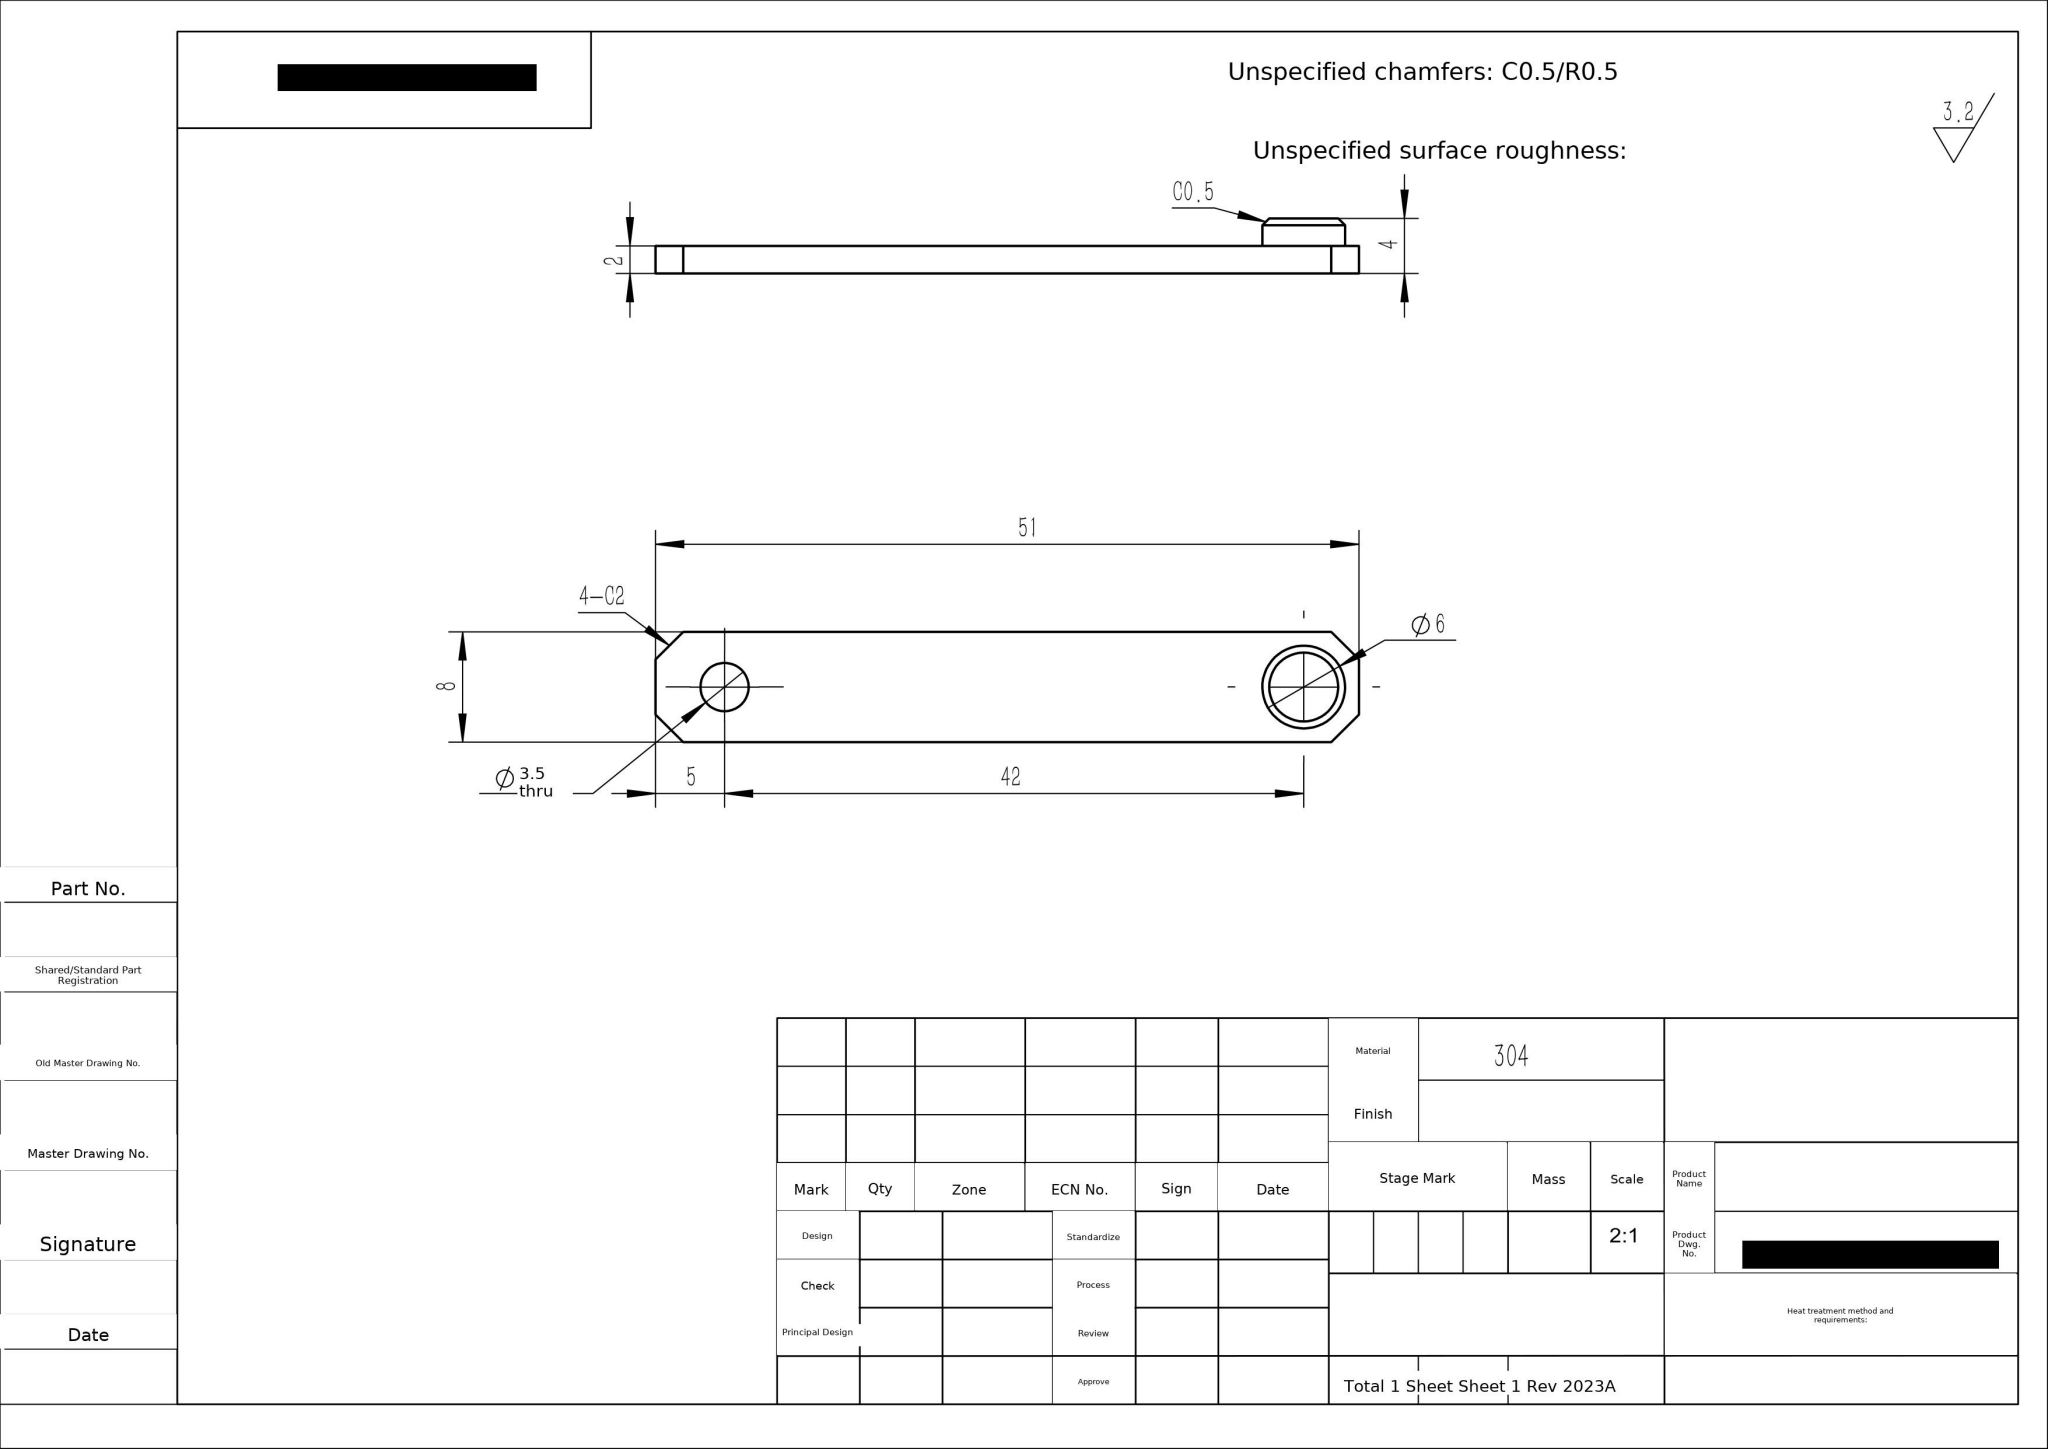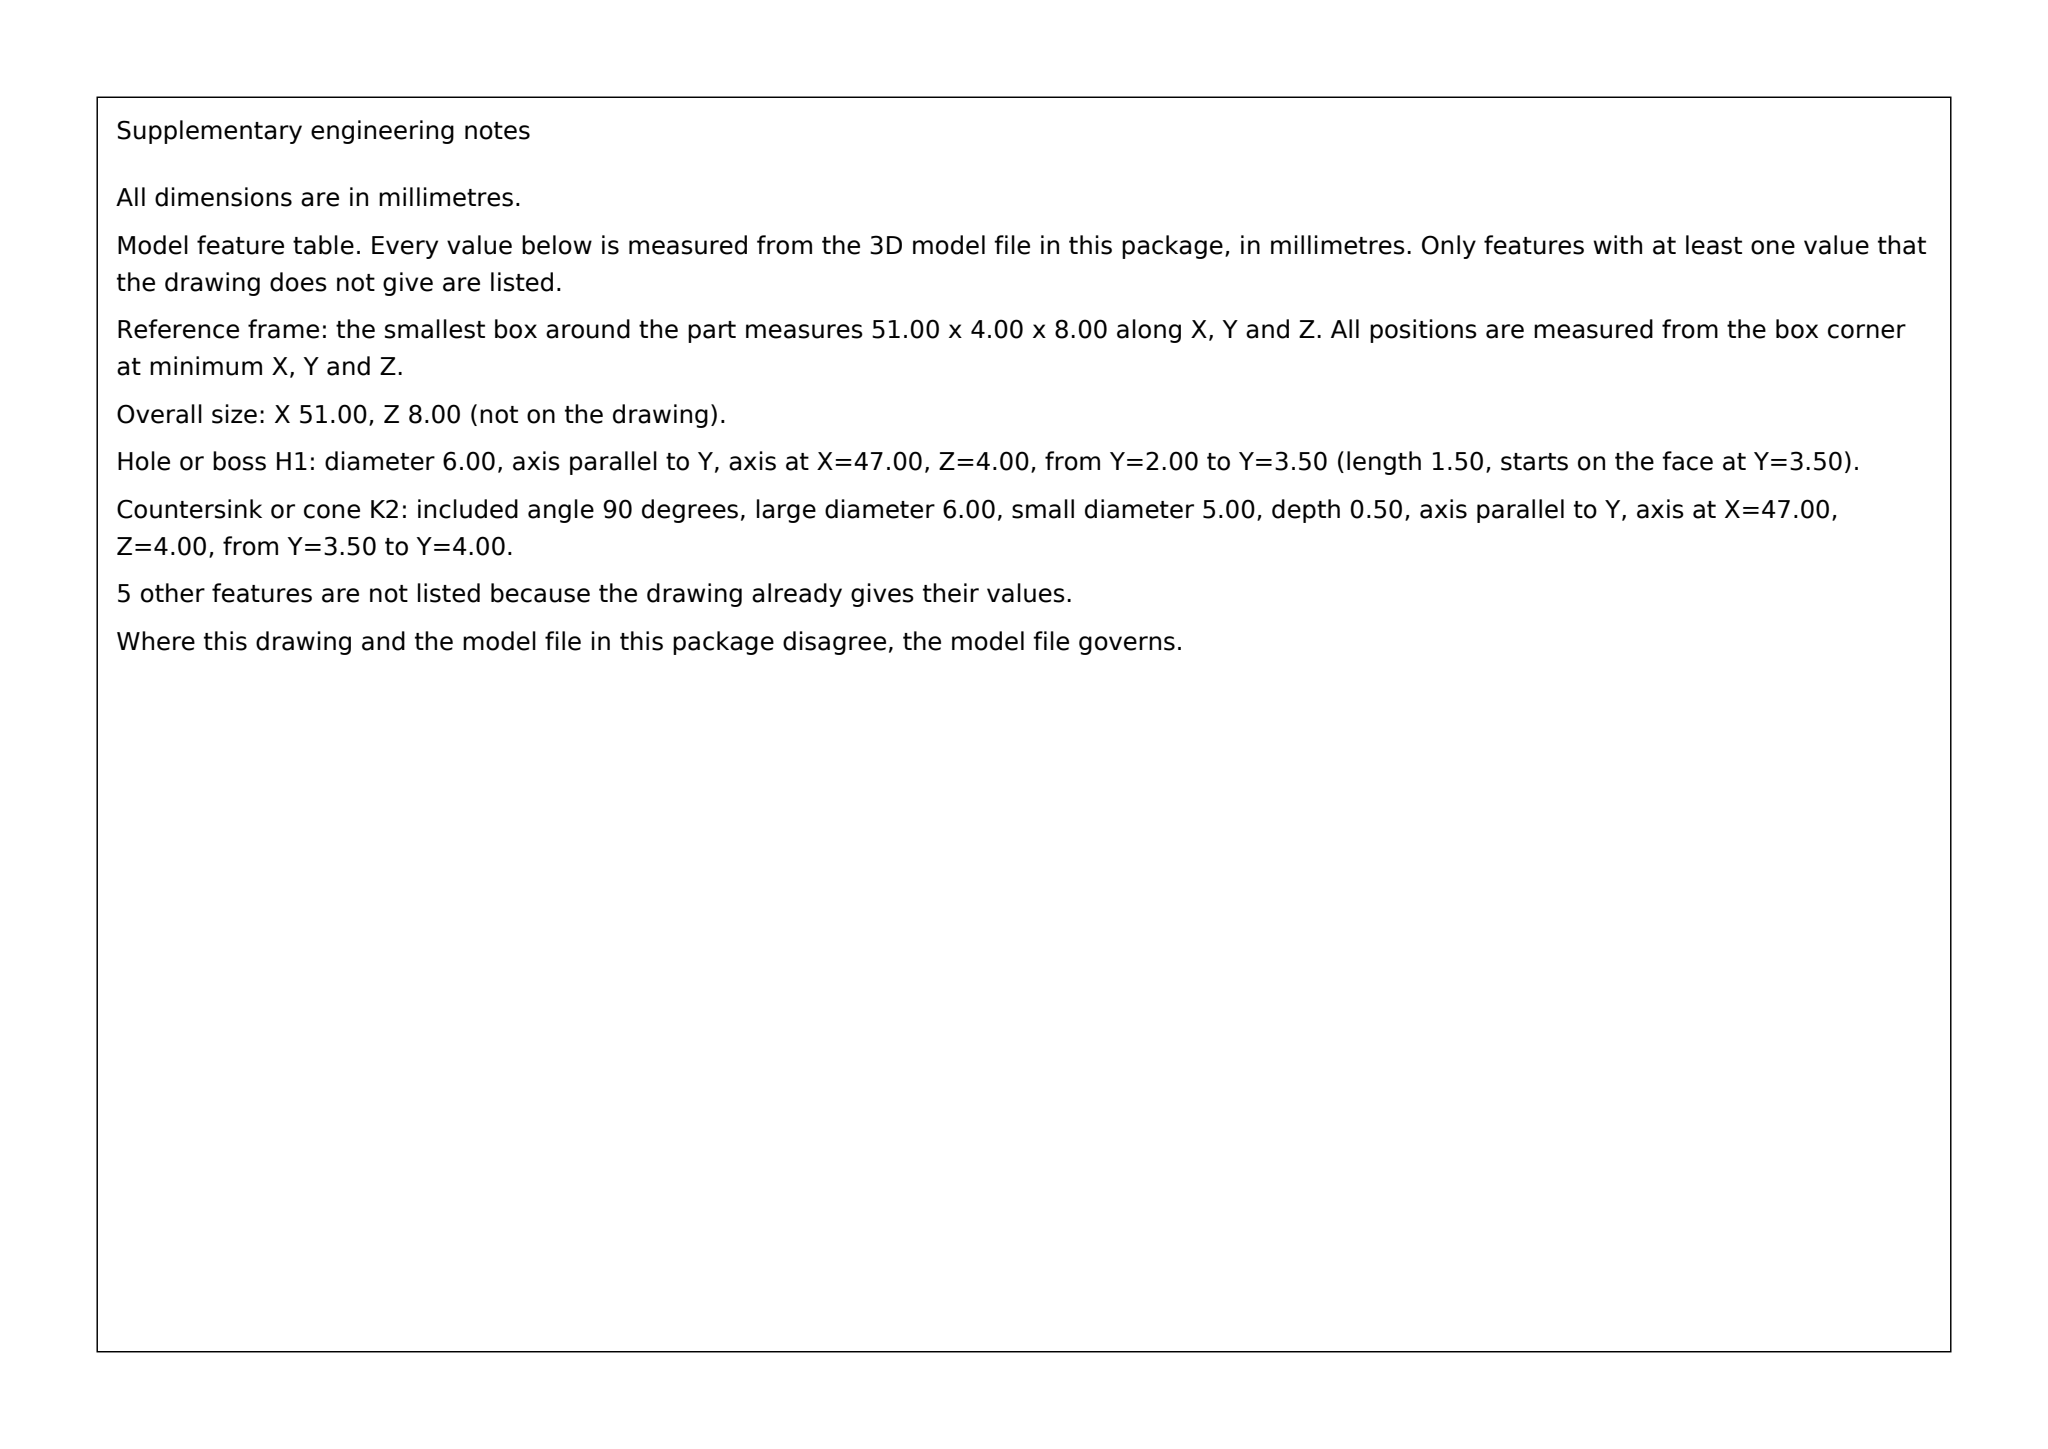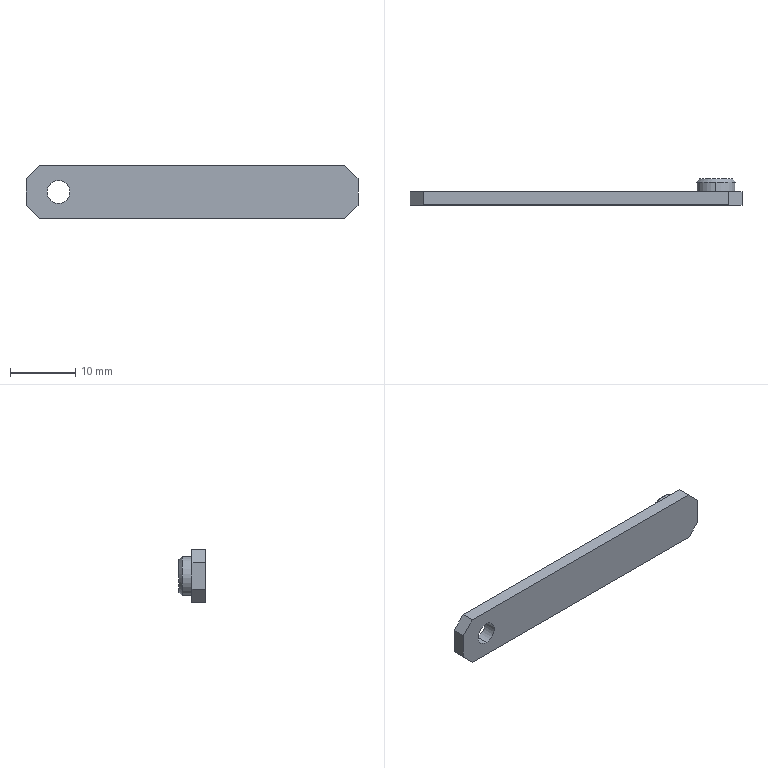Part | SolidWorks | mm | material 304 | 1 solid | 17 faces | box 51 x 4 x 8 mm | volume 835 mm3 | plane 11 | cylinder 4 | cone 2 | commonest cylinder face diameters 6 x2 3.5 x2
build123d program:
from build123d import *

# Parameters (mm, degrees)
SKETCH1_W           = 51
SKETCH1_H           = 8
BOSS_EXTRUDE1_DEPTH = 2
SKETCH2_R           = 1.75
CUT_EXTRUDE1_DEPTH  = 52.662
SKETCH3_R           = 3
BOSS_EXTRUDE2_DEPTH = 2
CHAMFER1_SIZE       = 0.5
CHAMFER2_SIZE       = 2


with BuildPart() as part:
    # Sketch1 → Boss-Extrude1 (new body)
    with BuildSketch(Plane(origin=(0, 0, 0), x_dir=(1, 0, 0), z_dir=(0, 1, 0))):
        with Locations((25.5, 4)):
            Rectangle(SKETCH1_W, SKETCH1_H)
    extrude(amount=BOSS_EXTRUDE1_DEPTH)

    # Sketch2 → Cut-Extrude1 (cut, through all)
    with BuildSketch(Plane(origin=(0, 2, 0), x_dir=(1, 0, 0), z_dir=(0, 1, 0))):
        with Locations(Location((5, 4, 0), (0, 0, 270))):
            Circle(SKETCH2_R)
    extrude(amount=-CUT_EXTRUDE1_DEPTH, mode=Mode.SUBTRACT)

    # Sketch3 → Boss-Extrude2 (add)
    with BuildSketch(Plane(origin=(0, 2, 0), x_dir=(1, 0, 0), z_dir=(0, 1, 0))):
        with Locations(Location((47, 4, 0), (0, 0, 270))):
            Circle(SKETCH3_R)
    extrude(amount=BOSS_EXTRUDE2_DEPTH)

    # Chamfer1
    chamfer1_edges = [part.edges().sort_by_distance(p)[0] for p in [
        (47, 4, -7),
    ]]
    chamfer(chamfer1_edges, length=CHAMFER1_SIZE)

    # Chamfer2
    chamfer2_edges = [part.edges().sort_by_distance(p)[0] for p in [
        (0, 1, -8),
        (51, 1, -8),
        (51, 1, 0),
        (0, 1, 0),
    ]]
    chamfer(chamfer2_edges, length=CHAMFER2_SIZE)


solid = part.part
STEP:
#1=CARTESIAN_POINT('',(47.,4.,-1.5));
#2=VERTEX_POINT('',#1);
#3=CARTESIAN_POINT('',(47.,4.,-6.5));
#4=VERTEX_POINT('',#3);
#5=CARTESIAN_POINT('',(47.,4.,-4.));
#6=DIRECTION('',(0.,1.,0.));
#7=DIRECTION('',(0.,0.,1.));
#8=AXIS2_PLACEMENT_3D('',#5,#6,#7);
#9=CIRCLE('',#8,2.5);
#10=EDGE_CURVE('',#2,#4,#9,.T.);
#11=ORIENTED_EDGE('',*,*,#10,.F.);
#12=CARTESIAN_POINT('',(47.,3.5,-1.));
#13=VERTEX_POINT('',#12);
#14=CARTESIAN_POINT('',(47.,4.,-1.5));
#15=DIRECTION('',(0.,-0.7071,0.7071));
#16=VECTOR('',#15,1000.);
#17=LINE('',#14,#16);
#18=EDGE_CURVE('',#2,#13,#17,.T.);
#19=ORIENTED_EDGE('',*,*,#18,.T.);
#20=CARTESIAN_POINT('',(47.,3.5,-7.));
#21=VERTEX_POINT('',#20);
#22=CARTESIAN_POINT('',(47.,3.5,-4.));
#23=DIRECTION('',(0.,-1.,0.));
#24=DIRECTION('',(0.,0.,1.));
#25=AXIS2_PLACEMENT_3D('',#22,#23,#24);
#26=CIRCLE('',#25,3.);
#27=EDGE_CURVE('',#21,#13,#26,.T.);
#28=ORIENTED_EDGE('',*,*,#27,.F.);
#29=CARTESIAN_POINT('',(47.,4.,-6.5));
#30=DIRECTION('',(0.,-0.7071,-0.7071));
#31=VECTOR('',#30,1000.);
#32=LINE('',#29,#31);
#33=EDGE_CURVE('',#4,#21,#32,.T.);
#34=ORIENTED_EDGE('',*,*,#33,.F.);
#35=EDGE_LOOP('',(#11,#19,#28,#34));
#36=FACE_OUTER_BOUND('',#35,.T.);
#37=CARTESIAN_POINT('',(47.,4.,-4.));
#38=DIRECTION('',(0.,-1.,0.));
#39=DIRECTION('',(0.,0.,-1.));
#40=AXIS2_PLACEMENT_3D('',#37,#38,#39);
#41=CONICAL_SURFACE('',#40,2.5,0.7854);
#42=ADVANCED_FACE('',(#36),#41,.T.);
#43=ORIENTED_EDGE('',*,*,#27,.T.);
#44=CARTESIAN_POINT('',(47.,2.,-1.));
#45=VERTEX_POINT('',#44);
#46=CARTESIAN_POINT('',(47.,4.,-1.));
#47=DIRECTION('',(0.,-1.,0.));
#48=VECTOR('',#47,1000.);
#49=LINE('',#46,#48);
#50=EDGE_CURVE('',#13,#45,#49,.T.);
#51=ORIENTED_EDGE('',*,*,#50,.T.);
#52=CARTESIAN_POINT('',(47.,2.,-7.));
#53=VERTEX_POINT('',#52);
#54=CARTESIAN_POINT('',(47.,2.,-4.));
#55=DIRECTION('',(0.,1.,0.));
#56=DIRECTION('',(0.,0.,1.));
#57=AXIS2_PLACEMENT_3D('',#54,#55,#56);
#58=CIRCLE('',#57,3.);
#59=EDGE_CURVE('',#45,#53,#58,.T.);
#60=ORIENTED_EDGE('',*,*,#59,.T.);
#61=CARTESIAN_POINT('',(47.,4.,-7.));
#62=DIRECTION('',(0.,-1.,0.));
#63=VECTOR('',#62,1000.);
#64=LINE('',#61,#63);
#65=EDGE_CURVE('',#21,#53,#64,.T.);
#66=ORIENTED_EDGE('',*,*,#65,.F.);
#67=EDGE_LOOP('',(#43,#51,#60,#66));
#68=FACE_OUTER_BOUND('',#67,.T.);
#69=CARTESIAN_POINT('',(47.,4.,-4.));
#70=DIRECTION('',(0.,-1.,0.));
#71=DIRECTION('',(0.,0.,-1.));
#72=AXIS2_PLACEMENT_3D('',#69,#70,#71);
#73=CYLINDRICAL_SURFACE('',#72,3.);
#74=ADVANCED_FACE('',(#68),#73,.T.);
#75=CARTESIAN_POINT('',(5.,0.,-5.75));
#76=VERTEX_POINT('',#75);
#77=CARTESIAN_POINT('',(5.,0.,-2.25));
#78=VERTEX_POINT('',#77);
#79=CARTESIAN_POINT('',(5.,0.,-4.));
#80=DIRECTION('',(0.,1.,0.));
#81=DIRECTION('',(0.,0.,1.));
#82=AXIS2_PLACEMENT_3D('',#79,#80,#81);
#83=CIRCLE('',#82,1.75);
#84=EDGE_CURVE('',#76,#78,#83,.T.);
#85=ORIENTED_EDGE('',*,*,#84,.F.);
#86=CARTESIAN_POINT('',(5.,2.,-5.75));
#87=VERTEX_POINT('',#86);
#88=CARTESIAN_POINT('',(5.,0.,-5.75));
#89=DIRECTION('',(0.,1.,0.));
#90=VECTOR('',#89,1000.);
#91=LINE('',#88,#90);
#92=EDGE_CURVE('',#76,#87,#91,.T.);
#93=ORIENTED_EDGE('',*,*,#92,.T.);
#94=CARTESIAN_POINT('',(5.,2.,-2.25));
#95=VERTEX_POINT('',#94);
#96=CARTESIAN_POINT('',(5.,2.,-4.));
#97=DIRECTION('',(0.,1.,0.));
#98=DIRECTION('',(0.,0.,1.));
#99=AXIS2_PLACEMENT_3D('',#96,#97,#98);
#100=CIRCLE('',#99,1.75);
#101=EDGE_CURVE('',#87,#95,#100,.T.);
#102=ORIENTED_EDGE('',*,*,#101,.T.);
#103=CARTESIAN_POINT('',(5.,0.,-2.25));
#104=DIRECTION('',(0.,1.,0.));
#105=VECTOR('',#104,1000.);
#106=LINE('',#103,#105);
#107=EDGE_CURVE('',#78,#95,#106,.T.);
#108=ORIENTED_EDGE('',*,*,#107,.F.);
#109=EDGE_LOOP('',(#85,#93,#102,#108));
#110=FACE_OUTER_BOUND('',#109,.T.);
#111=CARTESIAN_POINT('',(5.,0.,-4.));
#112=DIRECTION('',(0.,1.,0.));
#113=DIRECTION('',(0.,0.,1.));
#114=AXIS2_PLACEMENT_3D('',#111,#112,#113);
#115=CYLINDRICAL_SURFACE('',#114,1.75);
#116=ADVANCED_FACE('',(#110),#115,.F.);
#117=CARTESIAN_POINT('',(51.,2.,-2.));
#118=VERTEX_POINT('',#117);
#119=CARTESIAN_POINT('',(51.,2.,-6.));
#120=VERTEX_POINT('',#119);
#121=CARTESIAN_POINT('',(51.,2.,-8.));
#122=DIRECTION('',(0.,0.,-1.));
#123=VECTOR('',#122,1000.);
#124=LINE('',#121,#123);
#125=EDGE_CURVE('',#118,#120,#124,.T.);
#126=ORIENTED_EDGE('',*,*,#125,.T.);
#127=CARTESIAN_POINT('',(49.,2.,-8.));
#128=VERTEX_POINT('',#127);
#129=CARTESIAN_POINT('',(28.5,2.,-28.5));
#130=DIRECTION('',(-0.7071,0.,-0.7071));
#131=VECTOR('',#130,1000.);
#132=LINE('',#129,#131);
#133=EDGE_CURVE('',#120,#128,#132,.T.);
#134=ORIENTED_EDGE('',*,*,#133,.T.);
#135=CARTESIAN_POINT('',(2.,2.,-8.));
#136=VERTEX_POINT('',#135);
#137=CARTESIAN_POINT('',(0.,2.,-8.));
#138=DIRECTION('',(-1.,0.,0.));
#139=VECTOR('',#138,1000.);
#140=LINE('',#137,#139);
#141=EDGE_CURVE('',#128,#136,#140,.T.);
#142=ORIENTED_EDGE('',*,*,#141,.T.);
#143=CARTESIAN_POINT('',(0.,2.,-6.));
#144=VERTEX_POINT('',#143);
#145=CARTESIAN_POINT('',(-3.,2.,-3.));
#146=DIRECTION('',(-0.7071,0.,0.7071));
#147=VECTOR('',#146,1000.);
#148=LINE('',#145,#147);
#149=EDGE_CURVE('',#136,#144,#148,.T.);
#150=ORIENTED_EDGE('',*,*,#149,.T.);
#151=CARTESIAN_POINT('',(0.,2.,-2.));
#152=VERTEX_POINT('',#151);
#153=CARTESIAN_POINT('',(0.,2.,-8.));
#154=DIRECTION('',(-0.,0.,1.));
#155=VECTOR('',#154,1000.);
#156=LINE('',#153,#155);
#157=EDGE_CURVE('',#144,#152,#156,.T.);
#158=ORIENTED_EDGE('',*,*,#157,.T.);
#159=CARTESIAN_POINT('',(2.,2.,0.));
#160=VERTEX_POINT('',#159);
#161=CARTESIAN_POINT('',(1.,2.,-1.));
#162=DIRECTION('',(0.7071,0.,0.7071));
#163=VECTOR('',#162,1000.);
#164=LINE('',#161,#163);
#165=EDGE_CURVE('',#152,#160,#164,.T.);
#166=ORIENTED_EDGE('',*,*,#165,.T.);
#167=CARTESIAN_POINT('',(49.,2.,0.));
#168=VERTEX_POINT('',#167);
#169=CARTESIAN_POINT('',(0.,2.,0.));
#170=DIRECTION('',(1.,0.,0.));
#171=VECTOR('',#170,1000.);
#172=LINE('',#169,#171);
#173=EDGE_CURVE('',#160,#168,#172,.T.);
#174=ORIENTED_EDGE('',*,*,#173,.T.);
#175=CARTESIAN_POINT('',(24.5,2.,24.5));
#176=DIRECTION('',(0.7071,0.,-0.7071));
#177=VECTOR('',#176,1000.);
#178=LINE('',#175,#177);
#179=EDGE_CURVE('',#168,#118,#178,.T.);
#180=ORIENTED_EDGE('',*,*,#179,.T.);
#181=EDGE_LOOP('',(#126,#134,#142,#150,#158,#166,#174,#180));
#182=FACE_OUTER_BOUND('',#181,.T.);
#183=CARTESIAN_POINT('',(5.,2.,-4.));
#184=DIRECTION('',(0.,1.,0.));
#185=DIRECTION('',(0.,0.,1.));
#186=AXIS2_PLACEMENT_3D('',#183,#184,#185);
#187=CIRCLE('',#186,1.75);
#188=EDGE_CURVE('',#95,#87,#187,.T.);
#189=ORIENTED_EDGE('',*,*,#188,.F.);
#190=ORIENTED_EDGE('',*,*,#101,.F.);
#191=EDGE_LOOP('',(#189,#190));
#192=FACE_BOUND('',#191,.T.);
#193=CARTESIAN_POINT('',(47.,2.,-4.));
#194=DIRECTION('',(0.,1.,0.));
#195=DIRECTION('',(0.,0.,1.));
#196=AXIS2_PLACEMENT_3D('',#193,#194,#195);
#197=CIRCLE('',#196,3.);
#198=EDGE_CURVE('',#53,#45,#197,.T.);
#199=ORIENTED_EDGE('',*,*,#198,.F.);
#200=ORIENTED_EDGE('',*,*,#59,.F.);
#201=EDGE_LOOP('',(#199,#200));
#202=FACE_BOUND('',#201,.T.);
#203=CARTESIAN_POINT('',(0.,2.,0.));
#204=DIRECTION('',(0.,1.,0.));
#205=DIRECTION('',(0.,0.,1.));
#206=AXIS2_PLACEMENT_3D('',#203,#204,#205);
#207=PLANE('',#206);
#208=ADVANCED_FACE('',(#182,#192,#202),#207,.T.);
#209=CARTESIAN_POINT('',(0.,0.,-6.));
#210=VERTEX_POINT('',#209);
#211=CARTESIAN_POINT('',(0.,0.,-2.));
#212=VERTEX_POINT('',#211);
#213=CARTESIAN_POINT('',(0.,0.,-8.));
#214=DIRECTION('',(-0.,0.,1.));
#215=VECTOR('',#214,1000.);
#216=LINE('',#213,#215);
#217=EDGE_CURVE('',#210,#212,#216,.T.);
#218=ORIENTED_EDGE('',*,*,#217,.T.);
#219=CARTESIAN_POINT('',(0.,2.,-2.));
#220=DIRECTION('',(0.,1.,0.));
#221=VECTOR('',#220,1000.);
#222=LINE('',#219,#221);
#223=EDGE_CURVE('',#212,#152,#222,.T.);
#224=ORIENTED_EDGE('',*,*,#223,.T.);
#225=ORIENTED_EDGE('',*,*,#157,.F.);
#226=CARTESIAN_POINT('',(0.,2.,-6.));
#227=DIRECTION('',(0.,-1.,0.));
#228=VECTOR('',#227,1000.);
#229=LINE('',#226,#228);
#230=EDGE_CURVE('',#144,#210,#229,.T.);
#231=ORIENTED_EDGE('',*,*,#230,.T.);
#232=EDGE_LOOP('',(#218,#224,#225,#231));
#233=FACE_OUTER_BOUND('',#232,.T.);
#234=CARTESIAN_POINT('',(0.,2.,-8.));
#235=DIRECTION('',(1.,0.,0.));
#236=DIRECTION('',(0.,0.,-1.));
#237=AXIS2_PLACEMENT_3D('',#234,#235,#236);
#238=PLANE('',#237);
#239=ADVANCED_FACE('',(#233),#238,.F.);
#240=CARTESIAN_POINT('',(2.,0.,0.));
#241=VERTEX_POINT('',#240);
#242=CARTESIAN_POINT('',(49.,0.,0.));
#243=VERTEX_POINT('',#242);
#244=CARTESIAN_POINT('',(0.,0.,0.));
#245=DIRECTION('',(1.,0.,0.));
#246=VECTOR('',#245,1000.);
#247=LINE('',#244,#246);
#248=EDGE_CURVE('',#241,#243,#247,.T.);
#249=ORIENTED_EDGE('',*,*,#248,.T.);
#250=CARTESIAN_POINT('',(49.,2.,0.));
#251=DIRECTION('',(0.,1.,0.));
#252=VECTOR('',#251,1000.);
#253=LINE('',#250,#252);
#254=EDGE_CURVE('',#243,#168,#253,.T.);
#255=ORIENTED_EDGE('',*,*,#254,.T.);
#256=ORIENTED_EDGE('',*,*,#173,.F.);
#257=CARTESIAN_POINT('',(2.,2.,0.));
#258=DIRECTION('',(0.,-1.,0.));
#259=VECTOR('',#258,1000.);
#260=LINE('',#257,#259);
#261=EDGE_CURVE('',#160,#241,#260,.T.);
#262=ORIENTED_EDGE('',*,*,#261,.T.);
#263=EDGE_LOOP('',(#249,#255,#256,#262));
#264=FACE_OUTER_BOUND('',#263,.T.);
#265=CARTESIAN_POINT('',(0.,2.,0.));
#266=DIRECTION('',(0.,0.,-1.));
#267=DIRECTION('',(-1.,0.,0.));
#268=AXIS2_PLACEMENT_3D('',#265,#266,#267);
#269=PLANE('',#268);
#270=ADVANCED_FACE('',(#264),#269,.F.);
#271=CARTESIAN_POINT('',(51.,0.,-2.));
#272=VERTEX_POINT('',#271);
#273=CARTESIAN_POINT('',(51.,0.,-6.));
#274=VERTEX_POINT('',#273);
#275=CARTESIAN_POINT('',(51.,0.,-8.));
#276=DIRECTION('',(0.,0.,-1.));
#277=VECTOR('',#276,1000.);
#278=LINE('',#275,#277);
#279=EDGE_CURVE('',#272,#274,#278,.T.);
#280=ORIENTED_EDGE('',*,*,#279,.T.);
#281=CARTESIAN_POINT('',(51.,2.,-6.));
#282=DIRECTION('',(0.,1.,0.));
#283=VECTOR('',#282,1000.);
#284=LINE('',#281,#283);
#285=EDGE_CURVE('',#274,#120,#284,.T.);
#286=ORIENTED_EDGE('',*,*,#285,.T.);
#287=ORIENTED_EDGE('',*,*,#125,.F.);
#288=CARTESIAN_POINT('',(51.,2.,-2.));
#289=DIRECTION('',(0.,-1.,0.));
#290=VECTOR('',#289,1000.);
#291=LINE('',#288,#290);
#292=EDGE_CURVE('',#118,#272,#291,.T.);
#293=ORIENTED_EDGE('',*,*,#292,.T.);
#294=EDGE_LOOP('',(#280,#286,#287,#293));
#295=FACE_OUTER_BOUND('',#294,.T.);
#296=CARTESIAN_POINT('',(51.,2.,-8.));
#297=DIRECTION('',(-1.,0.,0.));
#298=DIRECTION('',(0.,0.,1.));
#299=AXIS2_PLACEMENT_3D('',#296,#297,#298);
#300=PLANE('',#299);
#301=ADVANCED_FACE('',(#295),#300,.F.);
#302=ORIENTED_EDGE('',*,*,#141,.F.);
#303=CARTESIAN_POINT('',(49.,0.,-8.));
#304=VERTEX_POINT('',#303);
#305=CARTESIAN_POINT('',(49.,2.,-8.));
#306=DIRECTION('',(0.,-1.,0.));
#307=VECTOR('',#306,1000.);
#308=LINE('',#305,#307);
#309=EDGE_CURVE('',#128,#304,#308,.T.);
#310=ORIENTED_EDGE('',*,*,#309,.T.);
#311=CARTESIAN_POINT('',(2.,0.,-8.));
#312=VERTEX_POINT('',#311);
#313=CARTESIAN_POINT('',(0.,0.,-8.));
#314=DIRECTION('',(-1.,0.,0.));
#315=VECTOR('',#314,1000.);
#316=LINE('',#313,#315);
#317=EDGE_CURVE('',#304,#312,#316,.T.);
#318=ORIENTED_EDGE('',*,*,#317,.T.);
#319=CARTESIAN_POINT('',(2.,2.,-8.));
#320=DIRECTION('',(0.,1.,0.));
#321=VECTOR('',#320,1000.);
#322=LINE('',#319,#321);
#323=EDGE_CURVE('',#312,#136,#322,.T.);
#324=ORIENTED_EDGE('',*,*,#323,.T.);
#325=EDGE_LOOP('',(#302,#310,#318,#324));
#326=FACE_OUTER_BOUND('',#325,.T.);
#327=CARTESIAN_POINT('',(0.,2.,-8.));
#328=DIRECTION('',(0.,0.,1.));
#329=DIRECTION('',(1.,0.,0.));
#330=AXIS2_PLACEMENT_3D('',#327,#328,#329);
#331=PLANE('',#330);
#332=ADVANCED_FACE('',(#326),#331,.F.);
#333=CARTESIAN_POINT('',(5.,0.,-4.));
#334=DIRECTION('',(0.,1.,0.));
#335=DIRECTION('',(0.,0.,1.));
#336=AXIS2_PLACEMENT_3D('',#333,#334,#335);
#337=CIRCLE('',#336,1.75);
#338=EDGE_CURVE('',#78,#76,#337,.T.);
#339=ORIENTED_EDGE('',*,*,#338,.T.);
#340=ORIENTED_EDGE('',*,*,#84,.T.);
#341=EDGE_LOOP('',(#339,#340));
#342=FACE_BOUND('',#341,.T.);
#343=ORIENTED_EDGE('',*,*,#317,.F.);
#344=CARTESIAN_POINT('',(49.,0.,-8.));
#345=DIRECTION('',(0.7071,0.,0.7071));
#346=VECTOR('',#345,1000.);
#347=LINE('',#344,#346);
#348=EDGE_CURVE('',#304,#274,#347,.T.);
#349=ORIENTED_EDGE('',*,*,#348,.T.);
#350=ORIENTED_EDGE('',*,*,#279,.F.);
#351=CARTESIAN_POINT('',(51.,0.,-2.));
#352=DIRECTION('',(-0.7071,0.,0.7071));
#353=VECTOR('',#352,1000.);
#354=LINE('',#351,#353);
#355=EDGE_CURVE('',#272,#243,#354,.T.);
#356=ORIENTED_EDGE('',*,*,#355,.T.);
#357=ORIENTED_EDGE('',*,*,#248,.F.);
#358=CARTESIAN_POINT('',(2.,0.,0.));
#359=DIRECTION('',(-0.7071,0.,-0.7071));
#360=VECTOR('',#359,1000.);
#361=LINE('',#358,#360);
#362=EDGE_CURVE('',#241,#212,#361,.T.);
#363=ORIENTED_EDGE('',*,*,#362,.T.);
#364=ORIENTED_EDGE('',*,*,#217,.F.);
#365=CARTESIAN_POINT('',(0.,0.,-6.));
#366=DIRECTION('',(0.7071,0.,-0.7071));
#367=VECTOR('',#366,1000.);
#368=LINE('',#365,#367);
#369=EDGE_CURVE('',#210,#312,#368,.T.);
#370=ORIENTED_EDGE('',*,*,#369,.T.);
#371=EDGE_LOOP('',(#343,#349,#350,#356,#357,#363,#364,#370));
#372=FACE_OUTER_BOUND('',#371,.T.);
#373=CARTESIAN_POINT('',(0.,0.,0.));
#374=DIRECTION('',(0.,1.,0.));
#375=DIRECTION('',(0.,0.,1.));
#376=AXIS2_PLACEMENT_3D('',#373,#374,#375);
#377=PLANE('',#376);
#378=ADVANCED_FACE('',(#342,#372),#377,.F.);
#379=ORIENTED_EDGE('',*,*,#92,.F.);
#380=ORIENTED_EDGE('',*,*,#338,.F.);
#381=ORIENTED_EDGE('',*,*,#107,.T.);
#382=ORIENTED_EDGE('',*,*,#188,.T.);
#383=EDGE_LOOP('',(#379,#380,#381,#382));
#384=FACE_OUTER_BOUND('',#383,.T.);
#385=CARTESIAN_POINT('',(5.,0.,-4.));
#386=DIRECTION('',(0.,1.,0.));
#387=DIRECTION('',(0.,0.,1.));
#388=AXIS2_PLACEMENT_3D('',#385,#386,#387);
#389=CYLINDRICAL_SURFACE('',#388,1.75);
#390=ADVANCED_FACE('',(#384),#389,.F.);
#391=ORIENTED_EDGE('',*,*,#50,.F.);
#392=CARTESIAN_POINT('',(47.,3.5,-4.));
#393=DIRECTION('',(0.,-1.,0.));
#394=DIRECTION('',(0.,0.,1.));
#395=AXIS2_PLACEMENT_3D('',#392,#393,#394);
#396=CIRCLE('',#395,3.);
#397=EDGE_CURVE('',#13,#21,#396,.T.);
#398=ORIENTED_EDGE('',*,*,#397,.T.);
#399=ORIENTED_EDGE('',*,*,#65,.T.);
#400=ORIENTED_EDGE('',*,*,#198,.T.);
#401=EDGE_LOOP('',(#391,#398,#399,#400));
#402=FACE_OUTER_BOUND('',#401,.T.);
#403=CARTESIAN_POINT('',(47.,4.,-4.));
#404=DIRECTION('',(0.,-1.,0.));
#405=DIRECTION('',(0.,0.,-1.));
#406=AXIS2_PLACEMENT_3D('',#403,#404,#405);
#407=CYLINDRICAL_SURFACE('',#406,3.);
#408=ADVANCED_FACE('',(#402),#407,.T.);
#409=CARTESIAN_POINT('',(47.,4.,-4.));
#410=DIRECTION('',(0.,1.,0.));
#411=DIRECTION('',(0.,0.,1.));
#412=AXIS2_PLACEMENT_3D('',#409,#410,#411);
#413=CIRCLE('',#412,2.5);
#414=EDGE_CURVE('',#4,#2,#413,.T.);
#415=ORIENTED_EDGE('',*,*,#414,.T.);
#416=ORIENTED_EDGE('',*,*,#10,.T.);
#417=EDGE_LOOP('',(#415,#416));
#418=FACE_OUTER_BOUND('',#417,.T.);
#419=CARTESIAN_POINT('',(47.,4.,-4.));
#420=DIRECTION('',(0.,1.,0.));
#421=DIRECTION('',(0.,0.,1.));
#422=AXIS2_PLACEMENT_3D('',#419,#420,#421);
#423=PLANE('',#422);
#424=ADVANCED_FACE('',(#418),#423,.T.);
#425=ORIENTED_EDGE('',*,*,#18,.F.);
#426=ORIENTED_EDGE('',*,*,#414,.F.);
#427=ORIENTED_EDGE('',*,*,#33,.T.);
#428=ORIENTED_EDGE('',*,*,#397,.F.);
#429=EDGE_LOOP('',(#425,#426,#427,#428));
#430=FACE_OUTER_BOUND('',#429,.T.);
#431=CARTESIAN_POINT('',(47.,4.,-4.));
#432=DIRECTION('',(0.,-1.,0.));
#433=DIRECTION('',(0.,0.,-1.));
#434=AXIS2_PLACEMENT_3D('',#431,#432,#433);
#435=CONICAL_SURFACE('',#434,2.5,0.7854);
#436=ADVANCED_FACE('',(#430),#435,.T.);
#437=ORIENTED_EDGE('',*,*,#133,.F.);
#438=ORIENTED_EDGE('',*,*,#285,.F.);
#439=ORIENTED_EDGE('',*,*,#348,.F.);
#440=ORIENTED_EDGE('',*,*,#309,.F.);
#441=EDGE_LOOP('',(#437,#438,#439,#440));
#442=FACE_OUTER_BOUND('',#441,.T.);
#443=CARTESIAN_POINT('',(49.,2.,-8.));
#444=DIRECTION('',(-0.7071,0.,0.7071));
#445=DIRECTION('',(0.,-1.,0.));
#446=AXIS2_PLACEMENT_3D('',#443,#444,#445);
#447=PLANE('',#446);
#448=ADVANCED_FACE('',(#442),#447,.F.);
#449=ORIENTED_EDGE('',*,*,#179,.F.);
#450=ORIENTED_EDGE('',*,*,#254,.F.);
#451=ORIENTED_EDGE('',*,*,#355,.F.);
#452=ORIENTED_EDGE('',*,*,#292,.F.);
#453=EDGE_LOOP('',(#449,#450,#451,#452));
#454=FACE_OUTER_BOUND('',#453,.T.);
#455=CARTESIAN_POINT('',(51.,2.,-2.));
#456=DIRECTION('',(-0.7071,0.,-0.7071));
#457=DIRECTION('',(0.,-1.,0.));
#458=AXIS2_PLACEMENT_3D('',#455,#456,#457);
#459=PLANE('',#458);
#460=ADVANCED_FACE('',(#454),#459,.F.);
#461=ORIENTED_EDGE('',*,*,#165,.F.);
#462=ORIENTED_EDGE('',*,*,#223,.F.);
#463=ORIENTED_EDGE('',*,*,#362,.F.);
#464=ORIENTED_EDGE('',*,*,#261,.F.);
#465=EDGE_LOOP('',(#461,#462,#463,#464));
#466=FACE_OUTER_BOUND('',#465,.T.);
#467=CARTESIAN_POINT('',(2.,2.,0.));
#468=DIRECTION('',(0.7071,0.,-0.7071));
#469=DIRECTION('',(0.,-1.,0.));
#470=AXIS2_PLACEMENT_3D('',#467,#468,#469);
#471=PLANE('',#470);
#472=ADVANCED_FACE('',(#466),#471,.F.);
#473=ORIENTED_EDGE('',*,*,#149,.F.);
#474=ORIENTED_EDGE('',*,*,#323,.F.);
#475=ORIENTED_EDGE('',*,*,#369,.F.);
#476=ORIENTED_EDGE('',*,*,#230,.F.);
#477=EDGE_LOOP('',(#473,#474,#475,#476));
#478=FACE_OUTER_BOUND('',#477,.T.);
#479=CARTESIAN_POINT('',(0.,2.,-6.));
#480=DIRECTION('',(0.7071,0.,0.7071));
#481=DIRECTION('',(0.,-1.,0.));
#482=AXIS2_PLACEMENT_3D('',#479,#480,#481);
#483=PLANE('',#482);
#484=ADVANCED_FACE('',(#478),#483,.F.);
#485=CLOSED_SHELL('',(#42,#74,#116,#208,#239,#270,#301,#332,#378,#390,#408,#424,#436,#448,#460,#472,#484));
#486=MANIFOLD_SOLID_BREP('',#485);
#487=CARTESIAN_POINT('',(0.,0.,0.));
#488=DIRECTION('',(0.,0.,1.));
#489=DIRECTION('',(1.,0.,0.));
#490=AXIS2_PLACEMENT_3D('',#487,#488,#489);
#491=(LENGTH_UNIT()NAMED_UNIT(*)SI_UNIT(.MILLI.,.METRE.));
#492=UNCERTAINTY_MEASURE_WITH_UNIT(LENGTH_MEASURE(0.00001),#491,'','');
#493=(NAMED_UNIT(*)PLANE_ANGLE_UNIT()SI_UNIT($,.RADIAN.));
#494=(NAMED_UNIT(*)SI_UNIT($,.STERADIAN.)SOLID_ANGLE_UNIT());
#495=(GEOMETRIC_REPRESENTATION_CONTEXT(3)GLOBAL_UNCERTAINTY_ASSIGNED_CONTEXT((#492))GLOBAL_UNIT_ASSIGNED_CONTEXT((#491,#493,#494))REPRESENTATION_CONTEXT('',''));
#496=ADVANCED_BREP_SHAPE_REPRESENTATION('',(#486,#490),#495);